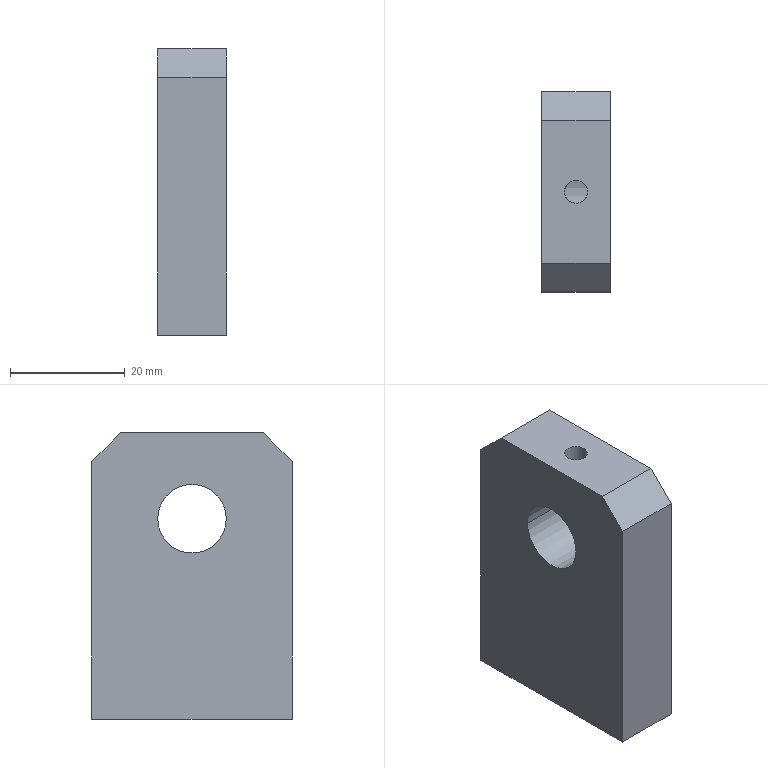Component | SolidWorks | SupportBase-1 | 1 solid | 24 faces | box 12 x 35 x 50 mm | volume 18827 mm3 | cone 8 | cylinder 8 | plane 8 | commonest cylinder face diameters 4.2 x4 4 x2 12 x2
build123d program:
from build123d import *

# Parameters (mm, degrees)
SKETCH1_W                      = 35
SKETCH1_H                      = 50
BOSS_EXTRUDE1_DEPTH            = 12
F_12_0_12_DIAMETER_HOLE1_D     = 12
F_4_0_4_DIAMETER_HOLE1_REACH   = 55.313
F_4_0_4_DIAMETER_HOLE1_BORE_R  = 2
F_4_2_4_2_DIAMETER_HOLE1_D     = 4.2
F_4_2_4_2_DIAMETER_HOLE1_DEPTH = 14
F_4_2_4_2_DIAMETER_HOLE1_TIP   = 1.262
CHAMFER1_SIZE                  = 0.425
CHAMFER2_SIZE                  = 5


with BuildPart() as part:
    # Sketch1 → Boss-Extrude1 (new body)
    with BuildSketch(Plane.XY.offset(6)):
        with Locations((0, -10)):
            Rectangle(SKETCH1_W, SKETCH1_H)
    extrude(amount=-BOSS_EXTRUDE1_DEPTH)

    # 12.0 _12_ Diameter Hole1 (through all)
    with Locations(Plane(origin=(0, 0, -6), x_dir=(-1, 0, 0), z_dir=(0, 0, -1))):
        with Locations((0, 0)):
            Hole(F_12_0_12_DIAMETER_HOLE1_D / 2)

    # 4.0 _4_ Diameter Hole1 bore → 4.0 _4_ Diameter Hole1 (cut, up to next)
    with BuildSketch(Plane(origin=(0, 15, 0), x_dir=(1, 0, 0), z_dir=(0, 1, 0)), mode=Mode.PRIVATE) as f_4_0_4_diameter_hole1_sk1:
        Circle(F_4_0_4_DIAMETER_HOLE1_BORE_R)
    f_4_0_4_diameter_hole1_tool1 = extrude(f_4_0_4_diameter_hole1_sk1.sketch, amount=-F_4_0_4_DIAMETER_HOLE1_REACH, mode=Mode.PRIVATE) & part.part
    add(f_4_0_4_diameter_hole1_tool1.solids().sort_by_distance((0, 15, 0))[0], mode=Mode.SUBTRACT)

    # 4.2 _4.2_ Diameter Hole1
    with Locations(Plane(origin=(0, -35, 0), x_dir=(-1, 0, 0), z_dir=(0, -1, 0))):
        with Locations((10, 0), (-10, 0)):
            Hole(F_4_2_4_2_DIAMETER_HOLE1_D / 2, depth=F_4_2_4_2_DIAMETER_HOLE1_DEPTH)
            with Locations((0, 0, -(F_4_2_4_2_DIAMETER_HOLE1_DEPTH + F_4_2_4_2_DIAMETER_HOLE1_TIP / 2))):  # 118° drill point
                Cone(0, F_4_2_4_2_DIAMETER_HOLE1_D / 2, F_4_2_4_2_DIAMETER_HOLE1_TIP, mode=Mode.SUBTRACT)

    # Chamfer1
    chamfer1_edges = [part.edges().sort_by_distance(p)[0] for p in [
        (7.9, -35, 0),
        (-12.1, -35, 0),
    ]]
    chamfer(chamfer1_edges, length=CHAMFER1_SIZE)

    # Chamfer2
    chamfer2_edges = [part.edges().sort_by_distance(p)[0] for p in [
        (-17.5, 15, 0),
        (17.5, 15, 0),
    ]]
    chamfer(chamfer2_edges, length=CHAMFER2_SIZE)


solid = part.part

# Placed as in the assembly
solid = solid.moved(Location((70, 556, -227.5), (90, -90, 0)))
STEP:
#1=COLOUR_RGB('',0.7922,0.8196,0.9333);
#2=FILL_AREA_STYLE_COLOUR('',#1);
#3=FILL_AREA_STYLE('',(#2));
#4=SURFACE_STYLE_FILL_AREA(#3);
#5=SURFACE_SIDE_STYLE('',(#4));
#6=SURFACE_STYLE_USAGE(.BOTH.,#5);
#7=PRESENTATION_STYLE_ASSIGNMENT((#6));
#8=CARTESIAN_POINT('',(2.673,21.496,-10.318));
#9=VERTEX_POINT('',#8);
#10=CARTESIAN_POINT('',(2.839,21.496,-10.318));
#11=VERTEX_POINT('',#10);
#12=CARTESIAN_POINT('',(2.756,21.496,-10.318));
#13=DIRECTION('',(-0.,-0.,-1.));
#14=DIRECTION('',(1.,0.,0.));
#15=AXIS2_PLACEMENT_3D('',#12,#13,#14);
#16=CIRCLE('',#15,0.08268);
#17=EDGE_CURVE('',#9,#11,#16,.T.);
#18=ORIENTED_EDGE('',*,*,#17,.F.);
#19=CARTESIAN_POINT('',(2.656,21.496,-10.335));
#20=VERTEX_POINT('',#19);
#21=CARTESIAN_POINT('',(2.673,21.496,-10.318));
#22=DIRECTION('',(-0.7071,-0.,-0.7071));
#23=VECTOR('',#22,39.37);
#24=LINE('',#21,#23);
#25=EDGE_CURVE('',#9,#20,#24,.T.);
#26=ORIENTED_EDGE('',*,*,#25,.T.);
#27=CARTESIAN_POINT('',(2.855,21.496,-10.335));
#28=VERTEX_POINT('',#27);
#29=CARTESIAN_POINT('',(2.756,21.496,-10.335));
#30=DIRECTION('',(0.,0.,1.));
#31=DIRECTION('',(1.,0.,0.));
#32=AXIS2_PLACEMENT_3D('',#29,#30,#31);
#33=CIRCLE('',#32,0.09941);
#34=EDGE_CURVE('',#28,#20,#33,.T.);
#35=ORIENTED_EDGE('',*,*,#34,.F.);
#36=CARTESIAN_POINT('',(2.839,21.496,-10.318));
#37=DIRECTION('',(0.7071,0.,-0.7071));
#38=VECTOR('',#37,39.37);
#39=LINE('',#36,#38);
#40=EDGE_CURVE('',#11,#28,#39,.T.);
#41=ORIENTED_EDGE('',*,*,#40,.F.);
#42=EDGE_LOOP('',(#18,#26,#35,#41));
#43=FACE_OUTER_BOUND('',#42,.T.);
#44=CARTESIAN_POINT('',(2.756,21.496,-10.318));
#45=DIRECTION('',(-0.,-0.,-1.));
#46=DIRECTION('',(1.,0.,0.));
#47=AXIS2_PLACEMENT_3D('',#44,#45,#46);
#48=CONICAL_SURFACE('',#47,0.08268,0.7854);
#49=ADVANCED_FACE('',(#43),#48,.F.);
#50=CARTESIAN_POINT('',(2.673,22.283,-10.318));
#51=VERTEX_POINT('',#50);
#52=CARTESIAN_POINT('',(2.839,22.283,-10.318));
#53=VERTEX_POINT('',#52);
#54=CARTESIAN_POINT('',(2.756,22.283,-10.318));
#55=DIRECTION('',(-0.,-0.,-1.));
#56=DIRECTION('',(1.,0.,0.));
#57=AXIS2_PLACEMENT_3D('',#54,#55,#56);
#58=CIRCLE('',#57,0.08268);
#59=EDGE_CURVE('',#51,#53,#58,.T.);
#60=ORIENTED_EDGE('',*,*,#59,.F.);
#61=CARTESIAN_POINT('',(2.656,22.283,-10.335));
#62=VERTEX_POINT('',#61);
#63=CARTESIAN_POINT('',(2.673,22.283,-10.318));
#64=DIRECTION('',(-0.7071,-0.,-0.7071));
#65=VECTOR('',#64,39.37);
#66=LINE('',#63,#65);
#67=EDGE_CURVE('',#51,#62,#66,.T.);
#68=ORIENTED_EDGE('',*,*,#67,.T.);
#69=CARTESIAN_POINT('',(2.855,22.283,-10.335));
#70=VERTEX_POINT('',#69);
#71=CARTESIAN_POINT('',(2.756,22.283,-10.335));
#72=DIRECTION('',(0.,0.,1.));
#73=DIRECTION('',(1.,0.,0.));
#74=AXIS2_PLACEMENT_3D('',#71,#72,#73);
#75=CIRCLE('',#74,0.09941);
#76=EDGE_CURVE('',#70,#62,#75,.T.);
#77=ORIENTED_EDGE('',*,*,#76,.F.);
#78=CARTESIAN_POINT('',(2.839,22.283,-10.318));
#79=DIRECTION('',(0.7071,0.,-0.7071));
#80=VECTOR('',#79,39.37);
#81=LINE('',#78,#80);
#82=EDGE_CURVE('',#53,#70,#81,.T.);
#83=ORIENTED_EDGE('',*,*,#82,.F.);
#84=EDGE_LOOP('',(#60,#68,#77,#83));
#85=FACE_OUTER_BOUND('',#84,.T.);
#86=CARTESIAN_POINT('',(2.756,22.283,-10.318));
#87=DIRECTION('',(-0.,-0.,-1.));
#88=DIRECTION('',(1.,0.,0.));
#89=AXIS2_PLACEMENT_3D('',#86,#87,#88);
#90=CONICAL_SURFACE('',#89,0.08268,0.7854);
#91=ADVANCED_FACE('',(#85),#90,.F.);
#92=CARTESIAN_POINT('',(2.673,22.283,-9.783));
#93=VERTEX_POINT('',#92);
#94=CARTESIAN_POINT('',(2.839,22.283,-9.783));
#95=VERTEX_POINT('',#94);
#96=CARTESIAN_POINT('',(2.756,22.283,-9.783));
#97=DIRECTION('',(-0.,-0.,-1.));
#98=DIRECTION('',(1.,0.,0.));
#99=AXIS2_PLACEMENT_3D('',#96,#97,#98);
#100=CIRCLE('',#99,0.08268);
#101=EDGE_CURVE('',#93,#95,#100,.T.);
#102=ORIENTED_EDGE('',*,*,#101,.F.);
#103=CARTESIAN_POINT('',(2.673,22.283,-10.335));
#104=DIRECTION('',(-0.,-0.,-1.));
#105=VECTOR('',#104,39.37);
#106=LINE('',#103,#105);
#107=EDGE_CURVE('',#93,#51,#106,.T.);
#108=ORIENTED_EDGE('',*,*,#107,.T.);
#109=ORIENTED_EDGE('',*,*,#59,.T.);
#110=CARTESIAN_POINT('',(2.839,22.283,-10.335));
#111=DIRECTION('',(-0.,-0.,-1.));
#112=VECTOR('',#111,39.37);
#113=LINE('',#110,#112);
#114=EDGE_CURVE('',#95,#53,#113,.T.);
#115=ORIENTED_EDGE('',*,*,#114,.F.);
#116=EDGE_LOOP('',(#102,#108,#109,#115));
#117=FACE_OUTER_BOUND('',#116,.T.);
#118=CARTESIAN_POINT('',(2.756,22.283,-10.335));
#119=DIRECTION('',(-0.,-0.,-1.));
#120=DIRECTION('',(1.,0.,0.));
#121=AXIS2_PLACEMENT_3D('',#118,#119,#120);
#122=CYLINDRICAL_SURFACE('',#121,0.08268);
#123=ADVANCED_FACE('',(#117),#122,.F.);
#124=CARTESIAN_POINT('',(2.756,22.283,-9.734));
#125=VERTEX_POINT('',#124);
#126=CARTESIAN_POINT('',(2.839,22.283,-9.783));
#127=DIRECTION('',(0.8572,0.,-0.515));
#128=VECTOR('',#127,39.37);
#129=LINE('',#126,#128);
#130=EDGE_CURVE('',#125,#95,#129,.T.);
#131=ORIENTED_EDGE('',*,*,#130,.F.);
#132=CARTESIAN_POINT('',(2.673,22.283,-9.783));
#133=DIRECTION('',(-0.8572,-0.,-0.515));
#134=VECTOR('',#133,39.37);
#135=LINE('',#132,#134);
#136=EDGE_CURVE('',#125,#93,#135,.T.);
#137=ORIENTED_EDGE('',*,*,#136,.T.);
#138=ORIENTED_EDGE('',*,*,#101,.T.);
#139=EDGE_LOOP('',(#131,#137,#138));
#140=FACE_OUTER_BOUND('',#139,.T.);
#141=CARTESIAN_POINT('',(2.756,22.283,-9.783));
#142=DIRECTION('',(-0.,-0.,-1.));
#143=DIRECTION('',(1.,0.,0.));
#144=AXIS2_PLACEMENT_3D('',#141,#142,#143);
#145=CONICAL_SURFACE('',#144,0.08268,1.03);
#146=ADVANCED_FACE('',(#140),#145,.F.);
#147=CARTESIAN_POINT('',(2.673,21.496,-9.783));
#148=VERTEX_POINT('',#147);
#149=CARTESIAN_POINT('',(2.839,21.496,-9.783));
#150=VERTEX_POINT('',#149);
#151=CARTESIAN_POINT('',(2.756,21.496,-9.783));
#152=DIRECTION('',(-0.,-0.,-1.));
#153=DIRECTION('',(1.,0.,0.));
#154=AXIS2_PLACEMENT_3D('',#151,#152,#153);
#155=CIRCLE('',#154,0.08268);
#156=EDGE_CURVE('',#148,#150,#155,.T.);
#157=ORIENTED_EDGE('',*,*,#156,.F.);
#158=CARTESIAN_POINT('',(2.673,21.496,-10.335));
#159=DIRECTION('',(-0.,-0.,-1.));
#160=VECTOR('',#159,39.37);
#161=LINE('',#158,#160);
#162=EDGE_CURVE('',#148,#9,#161,.T.);
#163=ORIENTED_EDGE('',*,*,#162,.T.);
#164=ORIENTED_EDGE('',*,*,#17,.T.);
#165=CARTESIAN_POINT('',(2.839,21.496,-10.335));
#166=DIRECTION('',(-0.,-0.,-1.));
#167=VECTOR('',#166,39.37);
#168=LINE('',#165,#167);
#169=EDGE_CURVE('',#150,#11,#168,.T.);
#170=ORIENTED_EDGE('',*,*,#169,.F.);
#171=EDGE_LOOP('',(#157,#163,#164,#170));
#172=FACE_OUTER_BOUND('',#171,.T.);
#173=CARTESIAN_POINT('',(2.756,21.496,-10.335));
#174=DIRECTION('',(-0.,-0.,-1.));
#175=DIRECTION('',(1.,0.,0.));
#176=AXIS2_PLACEMENT_3D('',#173,#174,#175);
#177=CYLINDRICAL_SURFACE('',#176,0.08268);
#178=ADVANCED_FACE('',(#172),#177,.F.);
#179=CARTESIAN_POINT('',(2.756,21.496,-9.734));
#180=VERTEX_POINT('',#179);
#181=CARTESIAN_POINT('',(2.839,21.496,-9.783));
#182=DIRECTION('',(0.8572,0.,-0.515));
#183=VECTOR('',#182,39.37);
#184=LINE('',#181,#183);
#185=EDGE_CURVE('',#180,#150,#184,.T.);
#186=ORIENTED_EDGE('',*,*,#185,.F.);
#187=CARTESIAN_POINT('',(2.673,21.496,-9.783));
#188=DIRECTION('',(-0.8572,-0.,-0.515));
#189=VECTOR('',#188,39.37);
#190=LINE('',#187,#189);
#191=EDGE_CURVE('',#180,#148,#190,.T.);
#192=ORIENTED_EDGE('',*,*,#191,.T.);
#193=ORIENTED_EDGE('',*,*,#156,.T.);
#194=EDGE_LOOP('',(#186,#192,#193));
#195=FACE_OUTER_BOUND('',#194,.T.);
#196=CARTESIAN_POINT('',(2.756,21.496,-9.783));
#197=DIRECTION('',(-0.,-0.,-1.));
#198=DIRECTION('',(1.,0.,0.));
#199=AXIS2_PLACEMENT_3D('',#196,#197,#198);
#200=CONICAL_SURFACE('',#199,0.08268,1.03);
#201=ADVANCED_FACE('',(#195),#200,.F.);
#202=CARTESIAN_POINT('',(2.835,21.89,-8.72));
#203=VERTEX_POINT('',#202);
#204=CARTESIAN_POINT('',(2.677,21.89,-8.72));
#205=VERTEX_POINT('',#204);
#206=CARTESIAN_POINT('',(2.835,21.89,-8.72));
#207=CARTESIAN_POINT('',(2.835,21.9,-8.72));
#208=CARTESIAN_POINT('',(2.833,21.911,-8.721));
#209=CARTESIAN_POINT('',(2.827,21.925,-8.723));
#210=CARTESIAN_POINT('',(2.824,21.929,-8.724));
#211=CARTESIAN_POINT('',(2.818,21.938,-8.725));
#212=CARTESIAN_POINT('',(2.815,21.942,-8.726));
#213=CARTESIAN_POINT('',(2.804,21.953,-8.729));
#214=CARTESIAN_POINT('',(2.796,21.958,-8.731));
#215=CARTESIAN_POINT('',(2.781,21.964,-8.733));
#216=CARTESIAN_POINT('',(2.776,21.966,-8.733));
#217=CARTESIAN_POINT('',(2.766,21.968,-8.734));
#218=CARTESIAN_POINT('',(2.761,21.969,-8.734));
#219=CARTESIAN_POINT('',(2.751,21.969,-8.734));
#220=CARTESIAN_POINT('',(2.746,21.968,-8.734));
#221=CARTESIAN_POINT('',(2.735,21.966,-8.733));
#222=CARTESIAN_POINT('',(2.73,21.964,-8.733));
#223=CARTESIAN_POINT('',(2.716,21.959,-8.731));
#224=CARTESIAN_POINT('',(2.707,21.953,-8.729));
#225=CARTESIAN_POINT('',(2.697,21.942,-8.726));
#226=CARTESIAN_POINT('',(2.693,21.938,-8.725));
#227=CARTESIAN_POINT('',(2.688,21.929,-8.724));
#228=CARTESIAN_POINT('',(2.685,21.925,-8.723));
#229=CARTESIAN_POINT('',(2.681,21.915,-8.722));
#230=CARTESIAN_POINT('',(2.68,21.91,-8.721));
#231=CARTESIAN_POINT('',(2.678,21.9,-8.721));
#232=CARTESIAN_POINT('',(2.677,21.895,-8.72));
#233=CARTESIAN_POINT('',(2.677,21.89,-8.72));
#234=B_SPLINE_CURVE_WITH_KNOTS('',3,(#206,#207,#208,#209,#210,#211,#212,#213,#214,#215,#216,#217,#218,#219,#220,#221,#222,#223,#224,#225,#226,#227,#228,#229,#230,#231,#232,#233),.UNSPECIFIED.,.F.,.F.,(4,2,2,2,2,2,2,2,2,2,2,2,2,4),(0.006298,0.007085,0.007479,0.007872,0.00866,0.009053,0.009447,0.00984,0.01023,0.01102,0.01141,0.01181,0.0122,0.0126),.UNSPECIFIED.);
#235=EDGE_CURVE('',#203,#205,#234,.T.);
#236=ORIENTED_EDGE('',*,*,#235,.F.);
#237=CARTESIAN_POINT('',(2.835,21.89,-8.366));
#238=VERTEX_POINT('',#237);
#239=CARTESIAN_POINT('',(2.835,21.89,-8.366));
#240=DIRECTION('',(0.,0.,1.));
#241=VECTOR('',#240,39.37);
#242=LINE('',#239,#241);
#243=EDGE_CURVE('',#203,#238,#242,.T.);
#244=ORIENTED_EDGE('',*,*,#243,.T.);
#245=CARTESIAN_POINT('',(2.677,21.89,-8.366));
#246=VERTEX_POINT('',#245);
#247=CARTESIAN_POINT('',(2.756,21.89,-8.366));
#248=DIRECTION('',(0.,0.,1.));
#249=DIRECTION('',(-1.,0.,0.));
#250=AXIS2_PLACEMENT_3D('',#247,#248,#249);
#251=CIRCLE('',#250,0.07874);
#252=EDGE_CURVE('',#238,#246,#251,.T.);
#253=ORIENTED_EDGE('',*,*,#252,.T.);
#254=CARTESIAN_POINT('',(2.677,21.89,-8.366));
#255=DIRECTION('',(0.,0.,1.));
#256=VECTOR('',#255,39.37);
#257=LINE('',#254,#256);
#258=EDGE_CURVE('',#205,#246,#257,.T.);
#259=ORIENTED_EDGE('',*,*,#258,.F.);
#260=EDGE_LOOP('',(#236,#244,#253,#259));
#261=FACE_OUTER_BOUND('',#260,.T.);
#262=CARTESIAN_POINT('',(2.756,21.89,-8.366));
#263=DIRECTION('',(0.,0.,1.));
#264=DIRECTION('',(-1.,0.,0.));
#265=AXIS2_PLACEMENT_3D('',#262,#263,#264);
#266=CYLINDRICAL_SURFACE('',#265,0.07874);
#267=ADVANCED_FACE('',(#261),#266,.F.);
#268=CARTESIAN_POINT('',(2.52,21.654,-8.957));
#269=VERTEX_POINT('',#268);
#270=CARTESIAN_POINT('',(2.52,22.126,-8.957));
#271=VERTEX_POINT('',#270);
#272=CARTESIAN_POINT('',(2.52,21.89,-8.957));
#273=DIRECTION('',(1.,0.,-0.));
#274=DIRECTION('',(0.,1.,0.));
#275=AXIS2_PLACEMENT_3D('',#272,#273,#274);
#276=CIRCLE('',#275,0.2362);
#277=EDGE_CURVE('',#269,#271,#276,.T.);
#278=ORIENTED_EDGE('',*,*,#277,.F.);
#279=CARTESIAN_POINT('',(2.992,21.654,-8.957));
#280=VERTEX_POINT('',#279);
#281=CARTESIAN_POINT('',(2.992,21.654,-8.957));
#282=DIRECTION('',(1.,0.,-0.));
#283=VECTOR('',#282,39.37);
#284=LINE('',#281,#283);
#285=EDGE_CURVE('',#269,#280,#284,.T.);
#286=ORIENTED_EDGE('',*,*,#285,.T.);
#287=CARTESIAN_POINT('',(2.992,22.126,-8.957));
#288=VERTEX_POINT('',#287);
#289=CARTESIAN_POINT('',(2.992,21.89,-8.957));
#290=DIRECTION('',(1.,0.,-0.));
#291=DIRECTION('',(0.,1.,0.));
#292=AXIS2_PLACEMENT_3D('',#289,#290,#291);
#293=CIRCLE('',#292,0.2362);
#294=EDGE_CURVE('',#280,#288,#293,.T.);
#295=ORIENTED_EDGE('',*,*,#294,.T.);
#296=CARTESIAN_POINT('',(2.992,22.126,-8.957));
#297=DIRECTION('',(1.,0.,-0.));
#298=VECTOR('',#297,39.37);
#299=LINE('',#296,#298);
#300=EDGE_CURVE('',#271,#288,#299,.T.);
#301=ORIENTED_EDGE('',*,*,#300,.F.);
#302=EDGE_LOOP('',(#278,#286,#295,#301));
#303=FACE_OUTER_BOUND('',#302,.T.);
#304=CARTESIAN_POINT('',(2.992,21.89,-8.957));
#305=DIRECTION('',(1.,0.,-0.));
#306=DIRECTION('',(0.,1.,0.));
#307=AXIS2_PLACEMENT_3D('',#304,#305,#306);
#308=CYLINDRICAL_SURFACE('',#307,0.2362);
#309=ADVANCED_FACE('',(#303),#308,.F.);
#310=ORIENTED_EDGE('',*,*,#76,.T.);
#311=CARTESIAN_POINT('',(2.756,22.283,-10.335));
#312=DIRECTION('',(0.,0.,1.));
#313=DIRECTION('',(1.,0.,0.));
#314=AXIS2_PLACEMENT_3D('',#311,#312,#313);
#315=CIRCLE('',#314,0.09941);
#316=EDGE_CURVE('',#62,#70,#315,.T.);
#317=ORIENTED_EDGE('',*,*,#316,.T.);
#318=EDGE_LOOP('',(#310,#317));
#319=FACE_BOUND('',#318,.T.);
#320=ORIENTED_EDGE('',*,*,#34,.T.);
#321=CARTESIAN_POINT('',(2.756,21.496,-10.335));
#322=DIRECTION('',(0.,0.,1.));
#323=DIRECTION('',(1.,0.,0.));
#324=AXIS2_PLACEMENT_3D('',#321,#322,#323);
#325=CIRCLE('',#324,0.09941);
#326=EDGE_CURVE('',#20,#28,#325,.T.);
#327=ORIENTED_EDGE('',*,*,#326,.T.);
#328=EDGE_LOOP('',(#320,#327));
#329=FACE_BOUND('',#328,.T.);
#330=CARTESIAN_POINT('',(2.52,22.579,-10.335));
#331=VERTEX_POINT('',#330);
#332=CARTESIAN_POINT('',(2.52,21.201,-10.335));
#333=VERTEX_POINT('',#332);
#334=CARTESIAN_POINT('',(2.52,22.579,-10.335));
#335=DIRECTION('',(0.,-1.,0.));
#336=VECTOR('',#335,39.37);
#337=LINE('',#334,#336);
#338=EDGE_CURVE('',#331,#333,#337,.T.);
#339=ORIENTED_EDGE('',*,*,#338,.F.);
#340=CARTESIAN_POINT('',(2.992,22.579,-10.335));
#341=VERTEX_POINT('',#340);
#342=CARTESIAN_POINT('',(2.992,22.579,-10.335));
#343=DIRECTION('',(-1.,-0.,0.));
#344=VECTOR('',#343,39.37);
#345=LINE('',#342,#344);
#346=EDGE_CURVE('',#341,#331,#345,.T.);
#347=ORIENTED_EDGE('',*,*,#346,.F.);
#348=CARTESIAN_POINT('',(2.992,21.201,-10.335));
#349=VERTEX_POINT('',#348);
#350=CARTESIAN_POINT('',(2.992,22.579,-10.335));
#351=DIRECTION('',(0.,-1.,0.));
#352=VECTOR('',#351,39.37);
#353=LINE('',#350,#352);
#354=EDGE_CURVE('',#341,#349,#353,.T.);
#355=ORIENTED_EDGE('',*,*,#354,.T.);
#356=CARTESIAN_POINT('',(2.992,21.201,-10.335));
#357=DIRECTION('',(-1.,-0.,0.));
#358=VECTOR('',#357,39.37);
#359=LINE('',#356,#358);
#360=EDGE_CURVE('',#349,#333,#359,.T.);
#361=ORIENTED_EDGE('',*,*,#360,.T.);
#362=EDGE_LOOP('',(#339,#347,#355,#361));
#363=FACE_OUTER_BOUND('',#362,.T.);
#364=CARTESIAN_POINT('',(2.992,22.579,-10.335));
#365=DIRECTION('',(-0.,-0.,-1.));
#366=DIRECTION('',(1.,0.,-0.));
#367=AXIS2_PLACEMENT_3D('',#364,#365,#366);
#368=PLANE('',#367);
#369=ADVANCED_FACE('',(#319,#329,#363),#368,.T.);
#370=CARTESIAN_POINT('',(2.52,22.579,-8.563));
#371=VERTEX_POINT('',#370);
#372=CARTESIAN_POINT('',(2.52,22.579,-8.366));
#373=DIRECTION('',(-0.,-0.,-1.));
#374=VECTOR('',#373,39.37);
#375=LINE('',#372,#374);
#376=EDGE_CURVE('',#371,#331,#375,.T.);
#377=ORIENTED_EDGE('',*,*,#376,.F.);
#378=CARTESIAN_POINT('',(2.992,22.579,-8.563));
#379=VERTEX_POINT('',#378);
#380=CARTESIAN_POINT('',(2.992,22.579,-8.563));
#381=DIRECTION('',(1.,0.,-0.));
#382=VECTOR('',#381,39.37);
#383=LINE('',#380,#382);
#384=EDGE_CURVE('',#371,#379,#383,.T.);
#385=ORIENTED_EDGE('',*,*,#384,.T.);
#386=CARTESIAN_POINT('',(2.992,22.579,-8.366));
#387=DIRECTION('',(-0.,-0.,-1.));
#388=VECTOR('',#387,39.37);
#389=LINE('',#386,#388);
#390=EDGE_CURVE('',#379,#341,#389,.T.);
#391=ORIENTED_EDGE('',*,*,#390,.T.);
#392=ORIENTED_EDGE('',*,*,#346,.T.);
#393=EDGE_LOOP('',(#377,#385,#391,#392));
#394=FACE_OUTER_BOUND('',#393,.T.);
#395=CARTESIAN_POINT('',(2.992,22.579,-8.366));
#396=DIRECTION('',(-0.,1.,-0.));
#397=DIRECTION('',(-1.,-0.,0.));
#398=AXIS2_PLACEMENT_3D('',#395,#396,#397);
#399=PLANE('',#398);
#400=ADVANCED_FACE('',(#394),#399,.T.);
#401=CARTESIAN_POINT('',(2.756,21.89,-8.366));
#402=DIRECTION('',(0.,0.,1.));
#403=DIRECTION('',(-1.,0.,0.));
#404=AXIS2_PLACEMENT_3D('',#401,#402,#403);
#405=CIRCLE('',#404,0.07874);
#406=EDGE_CURVE('',#246,#238,#405,.T.);
#407=ORIENTED_EDGE('',*,*,#406,.F.);
#408=ORIENTED_EDGE('',*,*,#252,.F.);
#409=EDGE_LOOP('',(#407,#408));
#410=FACE_BOUND('',#409,.T.);
#411=CARTESIAN_POINT('',(2.992,21.398,-8.366));
#412=VERTEX_POINT('',#411);
#413=CARTESIAN_POINT('',(2.992,22.382,-8.366));
#414=VERTEX_POINT('',#413);
#415=CARTESIAN_POINT('',(2.992,21.201,-8.366));
#416=DIRECTION('',(-0.,1.,-0.));
#417=VECTOR('',#416,39.37);
#418=LINE('',#415,#417);
#419=EDGE_CURVE('',#412,#414,#418,.T.);
#420=ORIENTED_EDGE('',*,*,#419,.T.);
#421=CARTESIAN_POINT('',(2.52,22.382,-8.366));
#422=VERTEX_POINT('',#421);
#423=CARTESIAN_POINT('',(2.992,22.382,-8.366));
#424=DIRECTION('',(-1.,-0.,0.));
#425=VECTOR('',#424,39.37);
#426=LINE('',#423,#425);
#427=EDGE_CURVE('',#414,#422,#426,.T.);
#428=ORIENTED_EDGE('',*,*,#427,.T.);
#429=CARTESIAN_POINT('',(2.52,21.398,-8.366));
#430=VERTEX_POINT('',#429);
#431=CARTESIAN_POINT('',(2.52,21.201,-8.366));
#432=DIRECTION('',(-0.,1.,-0.));
#433=VECTOR('',#432,39.37);
#434=LINE('',#431,#433);
#435=EDGE_CURVE('',#430,#422,#434,.T.);
#436=ORIENTED_EDGE('',*,*,#435,.F.);
#437=CARTESIAN_POINT('',(2.992,21.398,-8.366));
#438=DIRECTION('',(1.,0.,-0.));
#439=VECTOR('',#438,39.37);
#440=LINE('',#437,#439);
#441=EDGE_CURVE('',#430,#412,#440,.T.);
#442=ORIENTED_EDGE('',*,*,#441,.T.);
#443=EDGE_LOOP('',(#420,#428,#436,#442));
#444=FACE_OUTER_BOUND('',#443,.T.);
#445=CARTESIAN_POINT('',(2.992,21.201,-8.366));
#446=DIRECTION('',(0.,0.,1.));
#447=DIRECTION('',(-1.,-0.,0.));
#448=AXIS2_PLACEMENT_3D('',#445,#446,#447);
#449=PLANE('',#448);
#450=ADVANCED_FACE('',(#410,#444),#449,.T.);
#451=CARTESIAN_POINT('',(2.992,21.201,-8.563));
#452=VERTEX_POINT('',#451);
#453=CARTESIAN_POINT('',(2.992,21.201,-10.335));
#454=DIRECTION('',(0.,0.,1.));
#455=VECTOR('',#454,39.37);
#456=LINE('',#453,#455);
#457=EDGE_CURVE('',#349,#452,#456,.T.);
#458=ORIENTED_EDGE('',*,*,#457,.T.);
#459=CARTESIAN_POINT('',(2.52,21.201,-8.563));
#460=VERTEX_POINT('',#459);
#461=CARTESIAN_POINT('',(2.992,21.201,-8.563));
#462=DIRECTION('',(-1.,-0.,0.));
#463=VECTOR('',#462,39.37);
#464=LINE('',#461,#463);
#465=EDGE_CURVE('',#452,#460,#464,.T.);
#466=ORIENTED_EDGE('',*,*,#465,.T.);
#467=CARTESIAN_POINT('',(2.52,21.201,-10.335));
#468=DIRECTION('',(0.,0.,1.));
#469=VECTOR('',#468,39.37);
#470=LINE('',#467,#469);
#471=EDGE_CURVE('',#333,#460,#470,.T.);
#472=ORIENTED_EDGE('',*,*,#471,.F.);
#473=ORIENTED_EDGE('',*,*,#360,.F.);
#474=EDGE_LOOP('',(#458,#466,#472,#473));
#475=FACE_OUTER_BOUND('',#474,.T.);
#476=CARTESIAN_POINT('',(2.992,21.201,-10.335));
#477=DIRECTION('',(0.,-1.,0.));
#478=DIRECTION('',(1.,0.,-0.));
#479=AXIS2_PLACEMENT_3D('',#476,#477,#478);
#480=PLANE('',#479);
#481=ADVANCED_FACE('',(#475),#480,.T.);
#482=CARTESIAN_POINT('',(2.992,21.89,-8.957));
#483=DIRECTION('',(1.,0.,-0.));
#484=DIRECTION('',(0.,1.,0.));
#485=AXIS2_PLACEMENT_3D('',#482,#483,#484);
#486=CIRCLE('',#485,0.2362);
#487=EDGE_CURVE('',#288,#280,#486,.T.);
#488=ORIENTED_EDGE('',*,*,#487,.F.);
#489=ORIENTED_EDGE('',*,*,#294,.F.);
#490=EDGE_LOOP('',(#488,#489));
#491=FACE_BOUND('',#490,.T.);
#492=ORIENTED_EDGE('',*,*,#390,.F.);
#493=CARTESIAN_POINT('',(2.992,22.382,-8.366));
#494=DIRECTION('',(0.,-0.7071,0.7071));
#495=VECTOR('',#494,39.37);
#496=LINE('',#493,#495);
#497=EDGE_CURVE('',#379,#414,#496,.T.);
#498=ORIENTED_EDGE('',*,*,#497,.T.);
#499=ORIENTED_EDGE('',*,*,#419,.F.);
#500=CARTESIAN_POINT('',(2.992,21.201,-8.563));
#501=DIRECTION('',(-0.,-0.7071,-0.7071));
#502=VECTOR('',#501,39.37);
#503=LINE('',#500,#502);
#504=EDGE_CURVE('',#412,#452,#503,.T.);
#505=ORIENTED_EDGE('',*,*,#504,.T.);
#506=ORIENTED_EDGE('',*,*,#457,.F.);
#507=ORIENTED_EDGE('',*,*,#354,.F.);
#508=EDGE_LOOP('',(#492,#498,#499,#505,#506,#507));
#509=FACE_OUTER_BOUND('',#508,.T.);
#510=CARTESIAN_POINT('',(2.992,21.89,-8.957));
#511=DIRECTION('',(-1.,-0.,0.));
#512=DIRECTION('',(0.,-1.,0.));
#513=AXIS2_PLACEMENT_3D('',#510,#511,#512);
#514=PLANE('',#513);
#515=ADVANCED_FACE('',(#491,#509),#514,.F.);
#516=CARTESIAN_POINT('',(2.52,21.89,-8.957));
#517=DIRECTION('',(1.,0.,-0.));
#518=DIRECTION('',(0.,1.,0.));
#519=AXIS2_PLACEMENT_3D('',#516,#517,#518);
#520=CIRCLE('',#519,0.2362);
#521=EDGE_CURVE('',#271,#269,#520,.T.);
#522=ORIENTED_EDGE('',*,*,#521,.T.);
#523=ORIENTED_EDGE('',*,*,#277,.T.);
#524=EDGE_LOOP('',(#522,#523));
#525=FACE_BOUND('',#524,.T.);
#526=ORIENTED_EDGE('',*,*,#435,.T.);
#527=CARTESIAN_POINT('',(2.52,22.431,-8.415));
#528=DIRECTION('',(-0.,0.7071,-0.7071));
#529=VECTOR('',#528,39.37);
#530=LINE('',#527,#529);
#531=EDGE_CURVE('',#422,#371,#530,.T.);
#532=ORIENTED_EDGE('',*,*,#531,.T.);
#533=ORIENTED_EDGE('',*,*,#376,.T.);
#534=ORIENTED_EDGE('',*,*,#338,.T.);
#535=ORIENTED_EDGE('',*,*,#471,.T.);
#536=CARTESIAN_POINT('',(2.52,21.348,-8.415));
#537=DIRECTION('',(0.,0.7071,0.7071));
#538=VECTOR('',#537,39.37);
#539=LINE('',#536,#538);
#540=EDGE_CURVE('',#460,#430,#539,.T.);
#541=ORIENTED_EDGE('',*,*,#540,.T.);
#542=EDGE_LOOP('',(#526,#532,#533,#534,#535,#541));
#543=FACE_OUTER_BOUND('',#542,.T.);
#544=CARTESIAN_POINT('',(2.52,21.89,-8.957));
#545=DIRECTION('',(-1.,-0.,0.));
#546=DIRECTION('',(0.,-1.,0.));
#547=AXIS2_PLACEMENT_3D('',#544,#545,#546);
#548=PLANE('',#547);
#549=ADVANCED_FACE('',(#525,#543),#548,.T.);
#550=ORIENTED_EDGE('',*,*,#285,.F.);
#551=ORIENTED_EDGE('',*,*,#521,.F.);
#552=ORIENTED_EDGE('',*,*,#300,.T.);
#553=ORIENTED_EDGE('',*,*,#487,.T.);
#554=EDGE_LOOP('',(#550,#551,#552,#553));
#555=FACE_OUTER_BOUND('',#554,.T.);
#556=CARTESIAN_POINT('',(2.677,21.89,-8.72));
#557=CARTESIAN_POINT('',(2.677,21.885,-8.72));
#558=CARTESIAN_POINT('',(2.678,21.879,-8.721));
#559=CARTESIAN_POINT('',(2.68,21.869,-8.721));
#560=CARTESIAN_POINT('',(2.681,21.864,-8.722));
#561=CARTESIAN_POINT('',(2.685,21.855,-8.723));
#562=CARTESIAN_POINT('',(2.688,21.85,-8.724));
#563=CARTESIAN_POINT('',(2.693,21.842,-8.725));
#564=CARTESIAN_POINT('',(2.697,21.838,-8.726));
#565=CARTESIAN_POINT('',(2.707,21.827,-8.729));
#566=CARTESIAN_POINT('',(2.716,21.821,-8.731));
#567=CARTESIAN_POINT('',(2.73,21.815,-8.733));
#568=CARTESIAN_POINT('',(2.735,21.814,-8.733));
#569=CARTESIAN_POINT('',(2.746,21.812,-8.734));
#570=CARTESIAN_POINT('',(2.751,21.811,-8.734));
#571=CARTESIAN_POINT('',(2.761,21.811,-8.734));
#572=CARTESIAN_POINT('',(2.766,21.812,-8.734));
#573=CARTESIAN_POINT('',(2.776,21.814,-8.733));
#574=CARTESIAN_POINT('',(2.781,21.815,-8.733));
#575=CARTESIAN_POINT('',(2.791,21.819,-8.731));
#576=CARTESIAN_POINT('',(2.795,21.822,-8.731));
#577=CARTESIAN_POINT('',(2.804,21.827,-8.729));
#578=CARTESIAN_POINT('',(2.808,21.83,-8.728));
#579=CARTESIAN_POINT('',(2.815,21.838,-8.726));
#580=CARTESIAN_POINT('',(2.818,21.842,-8.725));
#581=CARTESIAN_POINT('',(2.824,21.85,-8.724));
#582=CARTESIAN_POINT('',(2.827,21.855,-8.723));
#583=CARTESIAN_POINT('',(2.831,21.864,-8.722));
#584=CARTESIAN_POINT('',(2.832,21.869,-8.721));
#585=CARTESIAN_POINT('',(2.834,21.879,-8.721));
#586=CARTESIAN_POINT('',(2.835,21.885,-8.72));
#587=CARTESIAN_POINT('',(2.835,21.89,-8.72));
#588=B_SPLINE_CURVE_WITH_KNOTS('',3,(#556,#557,#558,#559,#560,#561,#562,#563,#564,#565,#566,#567,#568,#569,#570,#571,#572,#573,#574,#575,#576,#577,#578,#579,#580,#581,#582,#583,#584,#585,#586,#587),.UNSPECIFIED.,.F.,.F.,(4,2,2,2,2,2,2,2,2,2,2,2,2,2,2,4),(0.,0.0003936,0.0007873,0.001181,0.001575,0.002362,0.002756,0.003149,0.003543,0.003936,0.00433,0.004724,0.005117,0.005511,0.005905,0.006298),.UNSPECIFIED.);
#589=EDGE_CURVE('',#205,#203,#588,.T.);
#590=ORIENTED_EDGE('',*,*,#589,.T.);
#591=ORIENTED_EDGE('',*,*,#235,.T.);
#592=EDGE_LOOP('',(#590,#591));
#593=FACE_BOUND('',#592,.T.);
#594=CARTESIAN_POINT('',(2.992,21.89,-8.957));
#595=DIRECTION('',(1.,0.,-0.));
#596=DIRECTION('',(0.,1.,0.));
#597=AXIS2_PLACEMENT_3D('',#594,#595,#596);
#598=CYLINDRICAL_SURFACE('',#597,0.2362);
#599=ADVANCED_FACE('',(#555,#593),#598,.F.);
#600=ORIENTED_EDGE('',*,*,#243,.F.);
#601=ORIENTED_EDGE('',*,*,#589,.F.);
#602=ORIENTED_EDGE('',*,*,#258,.T.);
#603=ORIENTED_EDGE('',*,*,#406,.T.);
#604=EDGE_LOOP('',(#600,#601,#602,#603));
#605=FACE_OUTER_BOUND('',#604,.T.);
#606=CARTESIAN_POINT('',(2.756,21.89,-8.366));
#607=DIRECTION('',(0.,0.,1.));
#608=DIRECTION('',(-1.,0.,0.));
#609=AXIS2_PLACEMENT_3D('',#606,#607,#608);
#610=CYLINDRICAL_SURFACE('',#609,0.07874);
#611=ADVANCED_FACE('',(#605),#610,.F.);
#612=ORIENTED_EDGE('',*,*,#191,.F.);
#613=ORIENTED_EDGE('',*,*,#185,.T.);
#614=CARTESIAN_POINT('',(2.756,21.496,-9.783));
#615=DIRECTION('',(-0.,-0.,-1.));
#616=DIRECTION('',(1.,0.,0.));
#617=AXIS2_PLACEMENT_3D('',#614,#615,#616);
#618=CIRCLE('',#617,0.08268);
#619=EDGE_CURVE('',#150,#148,#618,.T.);
#620=ORIENTED_EDGE('',*,*,#619,.T.);
#621=EDGE_LOOP('',(#612,#613,#620));
#622=FACE_OUTER_BOUND('',#621,.T.);
#623=CARTESIAN_POINT('',(2.756,21.496,-9.783));
#624=DIRECTION('',(-0.,-0.,-1.));
#625=DIRECTION('',(1.,0.,0.));
#626=AXIS2_PLACEMENT_3D('',#623,#624,#625);
#627=CONICAL_SURFACE('',#626,0.08268,1.03);
#628=ADVANCED_FACE('',(#622),#627,.F.);
#629=ORIENTED_EDGE('',*,*,#162,.F.);
#630=ORIENTED_EDGE('',*,*,#619,.F.);
#631=ORIENTED_EDGE('',*,*,#169,.T.);
#632=CARTESIAN_POINT('',(2.756,21.496,-10.318));
#633=DIRECTION('',(-0.,-0.,-1.));
#634=DIRECTION('',(1.,0.,0.));
#635=AXIS2_PLACEMENT_3D('',#632,#633,#634);
#636=CIRCLE('',#635,0.08268);
#637=EDGE_CURVE('',#11,#9,#636,.T.);
#638=ORIENTED_EDGE('',*,*,#637,.T.);
#639=EDGE_LOOP('',(#629,#630,#631,#638));
#640=FACE_OUTER_BOUND('',#639,.T.);
#641=CARTESIAN_POINT('',(2.756,21.496,-10.335));
#642=DIRECTION('',(-0.,-0.,-1.));
#643=DIRECTION('',(1.,0.,0.));
#644=AXIS2_PLACEMENT_3D('',#641,#642,#643);
#645=CYLINDRICAL_SURFACE('',#644,0.08268);
#646=ADVANCED_FACE('',(#640),#645,.F.);
#647=ORIENTED_EDGE('',*,*,#136,.F.);
#648=ORIENTED_EDGE('',*,*,#130,.T.);
#649=CARTESIAN_POINT('',(2.756,22.283,-9.783));
#650=DIRECTION('',(-0.,-0.,-1.));
#651=DIRECTION('',(1.,0.,0.));
#652=AXIS2_PLACEMENT_3D('',#649,#650,#651);
#653=CIRCLE('',#652,0.08268);
#654=EDGE_CURVE('',#95,#93,#653,.T.);
#655=ORIENTED_EDGE('',*,*,#654,.T.);
#656=EDGE_LOOP('',(#647,#648,#655));
#657=FACE_OUTER_BOUND('',#656,.T.);
#658=CARTESIAN_POINT('',(2.756,22.283,-9.783));
#659=DIRECTION('',(-0.,-0.,-1.));
#660=DIRECTION('',(1.,0.,0.));
#661=AXIS2_PLACEMENT_3D('',#658,#659,#660);
#662=CONICAL_SURFACE('',#661,0.08268,1.03);
#663=ADVANCED_FACE('',(#657),#662,.F.);
#664=ORIENTED_EDGE('',*,*,#107,.F.);
#665=ORIENTED_EDGE('',*,*,#654,.F.);
#666=ORIENTED_EDGE('',*,*,#114,.T.);
#667=CARTESIAN_POINT('',(2.756,22.283,-10.318));
#668=DIRECTION('',(-0.,-0.,-1.));
#669=DIRECTION('',(1.,0.,0.));
#670=AXIS2_PLACEMENT_3D('',#667,#668,#669);
#671=CIRCLE('',#670,0.08268);
#672=EDGE_CURVE('',#53,#51,#671,.T.);
#673=ORIENTED_EDGE('',*,*,#672,.T.);
#674=EDGE_LOOP('',(#664,#665,#666,#673));
#675=FACE_OUTER_BOUND('',#674,.T.);
#676=CARTESIAN_POINT('',(2.756,22.283,-10.335));
#677=DIRECTION('',(-0.,-0.,-1.));
#678=DIRECTION('',(1.,0.,0.));
#679=AXIS2_PLACEMENT_3D('',#676,#677,#678);
#680=CYLINDRICAL_SURFACE('',#679,0.08268);
#681=ADVANCED_FACE('',(#675),#680,.F.);
#682=ORIENTED_EDGE('',*,*,#67,.F.);
#683=ORIENTED_EDGE('',*,*,#672,.F.);
#684=ORIENTED_EDGE('',*,*,#82,.T.);
#685=ORIENTED_EDGE('',*,*,#316,.F.);
#686=EDGE_LOOP('',(#682,#683,#684,#685));
#687=FACE_OUTER_BOUND('',#686,.T.);
#688=CARTESIAN_POINT('',(2.756,22.283,-10.318));
#689=DIRECTION('',(-0.,-0.,-1.));
#690=DIRECTION('',(1.,0.,0.));
#691=AXIS2_PLACEMENT_3D('',#688,#689,#690);
#692=CONICAL_SURFACE('',#691,0.08268,0.7854);
#693=ADVANCED_FACE('',(#687),#692,.F.);
#694=ORIENTED_EDGE('',*,*,#25,.F.);
#695=ORIENTED_EDGE('',*,*,#637,.F.);
#696=ORIENTED_EDGE('',*,*,#40,.T.);
#697=ORIENTED_EDGE('',*,*,#326,.F.);
#698=EDGE_LOOP('',(#694,#695,#696,#697));
#699=FACE_OUTER_BOUND('',#698,.T.);
#700=CARTESIAN_POINT('',(2.756,21.496,-10.318));
#701=DIRECTION('',(-0.,-0.,-1.));
#702=DIRECTION('',(1.,0.,0.));
#703=AXIS2_PLACEMENT_3D('',#700,#701,#702);
#704=CONICAL_SURFACE('',#703,0.08268,0.7854);
#705=ADVANCED_FACE('',(#699),#704,.F.);
#706=ORIENTED_EDGE('',*,*,#497,.F.);
#707=ORIENTED_EDGE('',*,*,#384,.F.);
#708=ORIENTED_EDGE('',*,*,#531,.F.);
#709=ORIENTED_EDGE('',*,*,#427,.F.);
#710=EDGE_LOOP('',(#706,#707,#708,#709));
#711=FACE_OUTER_BOUND('',#710,.T.);
#712=CARTESIAN_POINT('',(2.992,22.382,-8.366));
#713=DIRECTION('',(-0.,-0.7071,-0.7071));
#714=DIRECTION('',(-1.,-0.,0.));
#715=AXIS2_PLACEMENT_3D('',#712,#713,#714);
#716=PLANE('',#715);
#717=ADVANCED_FACE('',(#711),#716,.F.);
#718=ORIENTED_EDGE('',*,*,#504,.F.);
#719=ORIENTED_EDGE('',*,*,#441,.F.);
#720=ORIENTED_EDGE('',*,*,#540,.F.);
#721=ORIENTED_EDGE('',*,*,#465,.F.);
#722=EDGE_LOOP('',(#718,#719,#720,#721));
#723=FACE_OUTER_BOUND('',#722,.T.);
#724=CARTESIAN_POINT('',(2.992,21.201,-8.563));
#725=DIRECTION('',(-0.,0.7071,-0.7071));
#726=DIRECTION('',(-1.,-0.,0.));
#727=AXIS2_PLACEMENT_3D('',#724,#725,#726);
#728=PLANE('',#727);
#729=ADVANCED_FACE('',(#723),#728,.F.);
#730=CLOSED_SHELL('',(#49,#91,#123,#146,#178,#201,#267,#309,#369,#400,#450,#481,#515,#549,#599,#611,#628,#646,#663,#681,#693,#705,#717,#729));
#731=MANIFOLD_SOLID_BREP('',#730);
#732=STYLED_ITEM('',(#7),#731);
#733=PRESENTATION_LAYER_ASSIGNMENT('','',(#732));
#734=CARTESIAN_POINT('',(0.,0.,0.));
#735=DIRECTION('',(0.,0.,1.));
#736=DIRECTION('',(1.,0.,0.));
#737=AXIS2_PLACEMENT_3D('',#734,#735,#736);
#738=(LENGTH_UNIT()NAMED_UNIT(*)SI_UNIT($,.METRE.));
#739=LENGTH_MEASURE_WITH_UNIT(LENGTH_MEASURE(0.0254),#738);
#740=DIMENSIONAL_EXPONENTS(1.,0.,0.,0.,0.,0.,0.);
#741=(CONVERSION_BASED_UNIT('',#739)LENGTH_UNIT()NAMED_UNIT(#740));
#742=UNCERTAINTY_MEASURE_WITH_UNIT(LENGTH_MEASURE(0.00001),#741,'','');
#743=(NAMED_UNIT(*)PLANE_ANGLE_UNIT()SI_UNIT($,.RADIAN.));
#744=(NAMED_UNIT(*)SI_UNIT($,.STERADIAN.)SOLID_ANGLE_UNIT());
#745=(GEOMETRIC_REPRESENTATION_CONTEXT(3)GLOBAL_UNCERTAINTY_ASSIGNED_CONTEXT((#742))GLOBAL_UNIT_ASSIGNED_CONTEXT((#741,#743,#744))REPRESENTATION_CONTEXT('',''));
#746=ADVANCED_BREP_SHAPE_REPRESENTATION('',(#731,#737),#745);
#747=(LENGTH_UNIT()NAMED_UNIT(*)SI_UNIT($,.METRE.));
#748=LENGTH_MEASURE_WITH_UNIT(LENGTH_MEASURE(0.0254),#747);
#749=DIMENSIONAL_EXPONENTS(1.,0.,0.,0.,0.,0.,0.);
#750=(CONVERSION_BASED_UNIT('',#748)LENGTH_UNIT()NAMED_UNIT(#749));
#751=UNCERTAINTY_MEASURE_WITH_UNIT(LENGTH_MEASURE(0.00001),#750,'','');
#752=(NAMED_UNIT(*)PLANE_ANGLE_UNIT()SI_UNIT($,.RADIAN.));
#753=(NAMED_UNIT(*)SI_UNIT($,.STERADIAN.)SOLID_ANGLE_UNIT());
#754=(GEOMETRIC_REPRESENTATION_CONTEXT(3)GLOBAL_UNCERTAINTY_ASSIGNED_CONTEXT((#751))GLOBAL_UNIT_ASSIGNED_CONTEXT((#750,#752,#753))REPRESENTATION_CONTEXT('',''));
#755=MECHANICAL_DESIGN_GEOMETRIC_PRESENTATION_REPRESENTATION('',(#732),#754);